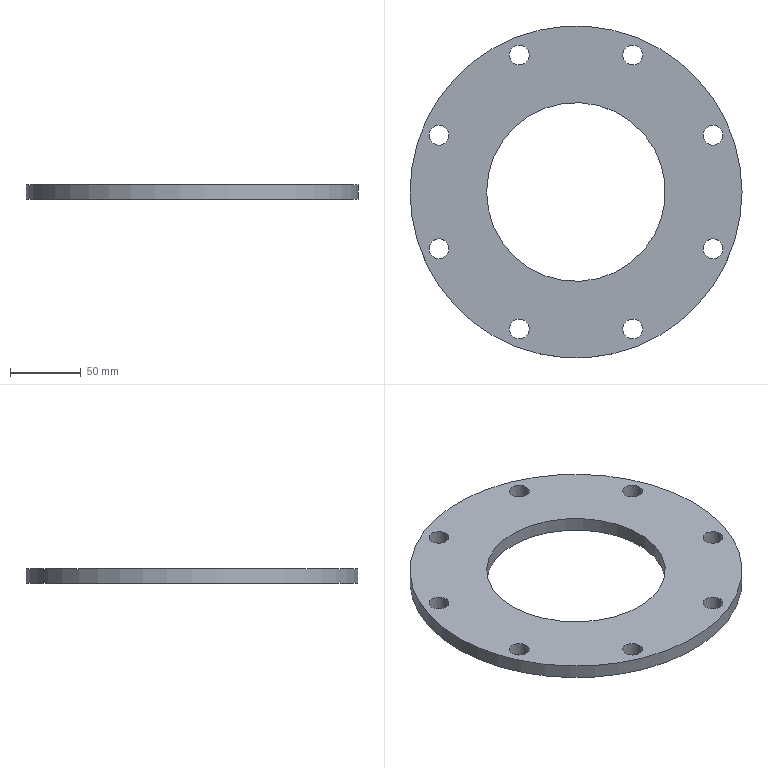Component | NX | CH3404_9-3 | 1 solid | 16 faces | volume 282838 mm3 | cylinder 12 | plane 4 | commonest cylinder face diameters 14 x8 234 x1 126 x1 150 x1 161 x1